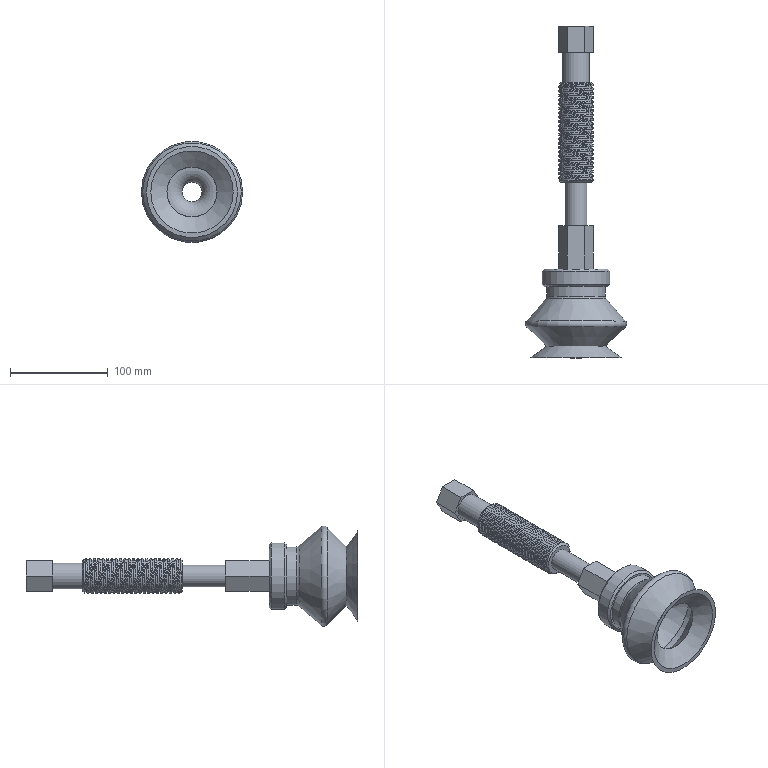Component | NX | A_SUCTION_CUP | 1 solid | 45 faces | volume 242855 mm3 | plane 21 | cone 10 | cylinder 9 | torus 3 | spline 2 | commonest cylinder face diameters 26.667 x1 52.978 x1 91.991 x1 60.254 x1 69.056 x1 33.53 x1 35.752 x1 22.222 x1